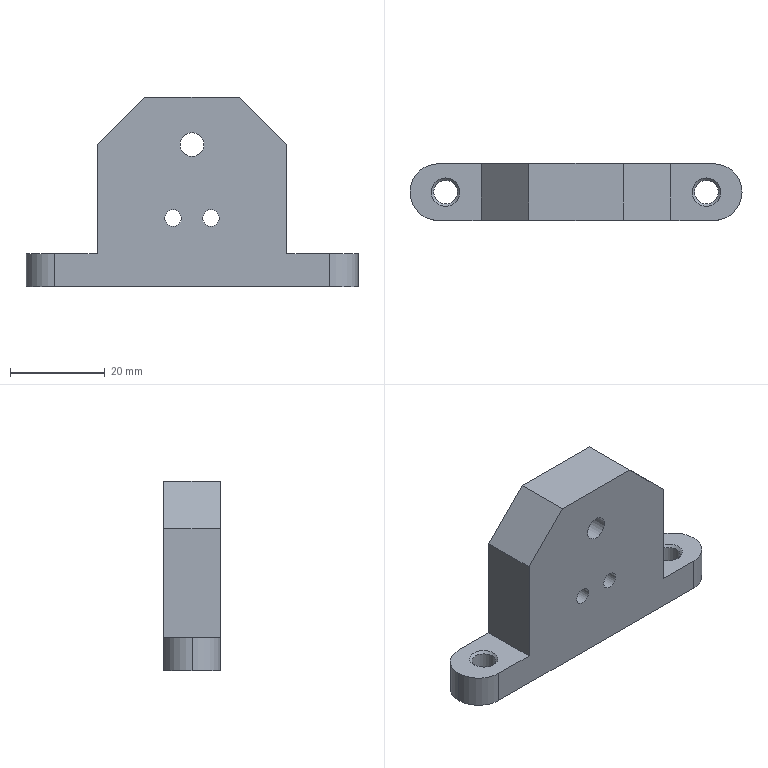Component | NX | SUPPORT_FRAME | 1 solid | 25 faces | volume 19222 mm3 | plane 12 | cylinder 11 | cone 2 | commonest cylinder face diameters 12 x4 5 x3 3.5 x2 6 x2